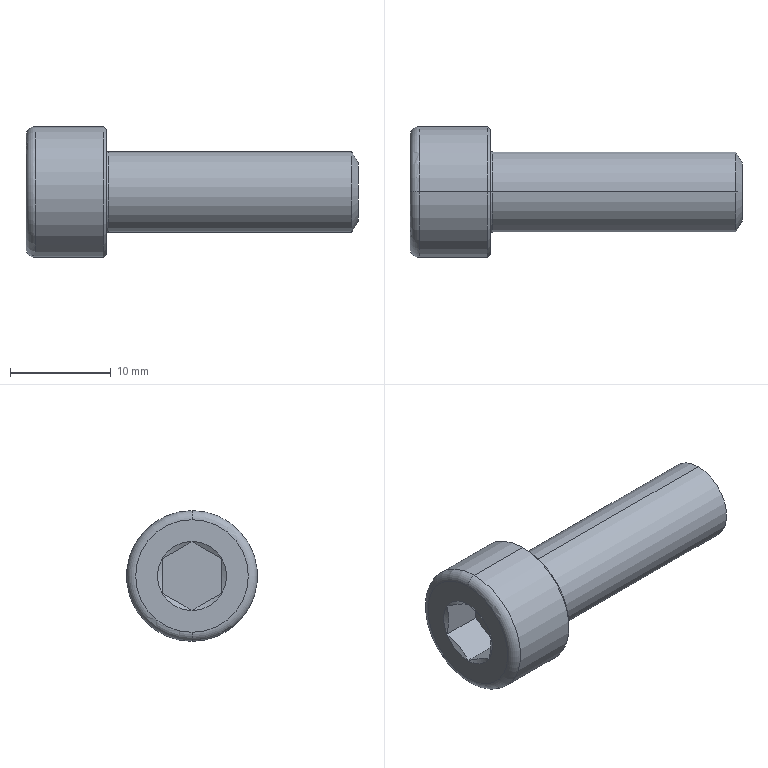Component | SolidWorks | M8_25_T70.1-1 | 1 solid | 28 faces | box 33 x 13 x 13 mm | volume 2179 mm3 | cone 10 | plane 10 | torus 4 | cylinder 4 | commonest cylinder face diameters 13 x2 8 x2 | material Plain Carbon Steel
STEP:
#1=COLOUR_RGB('',0.7922,0.8196,0.9333);
#2=FILL_AREA_STYLE_COLOUR('',#1);
#3=FILL_AREA_STYLE('',(#2));
#4=SURFACE_STYLE_FILL_AREA(#3);
#5=SURFACE_SIDE_STYLE('',(#4));
#6=SURFACE_STYLE_USAGE(.BOTH.,#5);
#7=PRESENTATION_STYLE_ASSIGNMENT((#6));
#8=CARTESIAN_POINT('',(-0.6339,1.67,1.426));
#9=VERTEX_POINT('',#8);
#10=CARTESIAN_POINT('',(-0.6339,1.67,1.914));
#11=VERTEX_POINT('',#10);
#12=CARTESIAN_POINT('',(-0.6339,1.67,1.67));
#13=DIRECTION('',(1.,0.,0.));
#14=DIRECTION('',(0.,0.,1.));
#15=AXIS2_PLACEMENT_3D('',#12,#13,#14);
#16=CIRCLE('',#15,0.2441);
#17=EDGE_CURVE('',#9,#11,#16,.T.);
#18=ORIENTED_EDGE('',*,*,#17,.F.);
#19=CARTESIAN_POINT('',(-0.6457,1.67,1.414));
#20=VERTEX_POINT('',#19);
#21=CARTESIAN_POINT('',(-0.6457,1.67,1.414));
#22=DIRECTION('',(-0.7071,0.,-0.7071));
#23=VECTOR('',#22,39.37);
#24=LINE('',#21,#23);
#25=EDGE_CURVE('',#9,#20,#24,.T.);
#26=ORIENTED_EDGE('',*,*,#25,.T.);
#27=CARTESIAN_POINT('',(-0.6457,1.67,1.926));
#28=VERTEX_POINT('',#27);
#29=CARTESIAN_POINT('',(-0.6457,1.67,1.67));
#30=DIRECTION('',(-1.,0.,0.));
#31=DIRECTION('',(0.,0.,1.));
#32=AXIS2_PLACEMENT_3D('',#29,#30,#31);
#33=CIRCLE('',#32,0.2559);
#34=EDGE_CURVE('',#28,#20,#33,.T.);
#35=ORIENTED_EDGE('',*,*,#34,.F.);
#36=CARTESIAN_POINT('',(-0.6457,1.67,1.926));
#37=DIRECTION('',(-0.7071,0.,0.7071));
#38=VECTOR('',#37,39.37);
#39=LINE('',#36,#38);
#40=EDGE_CURVE('',#11,#28,#39,.T.);
#41=ORIENTED_EDGE('',*,*,#40,.F.);
#42=EDGE_LOOP('',(#18,#26,#35,#41));
#43=FACE_OUTER_BOUND('',#42,.T.);
#44=CARTESIAN_POINT('',(-0.6457,1.67,1.67));
#45=DIRECTION('',(-1.,0.,0.));
#46=DIRECTION('',(0.,0.,1.));
#47=AXIS2_PLACEMENT_3D('',#44,#45,#46);
#48=CONICAL_SURFACE('',#47,0.2559,0.7854);
#49=ADVANCED_FACE('',(#43),#48,.T.);
#50=CARTESIAN_POINT('',(-0.9488,1.67,1.891));
#51=VERTEX_POINT('',#50);
#52=CARTESIAN_POINT('',(-0.9488,1.67,1.45));
#53=VERTEX_POINT('',#52);
#54=CARTESIAN_POINT('',(-0.9488,1.67,1.67));
#55=DIRECTION('',(-1.,0.,0.));
#56=DIRECTION('',(0.,0.,-1.));
#57=AXIS2_PLACEMENT_3D('',#54,#55,#56);
#58=CIRCLE('',#57,0.2205);
#59=EDGE_CURVE('',#51,#53,#58,.T.);
#60=ORIENTED_EDGE('',*,*,#59,.F.);
#61=CARTESIAN_POINT('',(-0.9134,1.67,1.926));
#62=VERTEX_POINT('',#61);
#63=CARTESIAN_POINT('',(-0.9134,1.67,1.891));
#64=DIRECTION('',(0.,1.,-0.));
#65=DIRECTION('',(0.,0.,1.));
#66=AXIS2_PLACEMENT_3D('',#63,#64,#65);
#67=CIRCLE('',#66,0.03543);
#68=EDGE_CURVE('',#51,#62,#67,.T.);
#69=ORIENTED_EDGE('',*,*,#68,.T.);
#70=CARTESIAN_POINT('',(-0.9134,1.67,1.414));
#71=VERTEX_POINT('',#70);
#72=CARTESIAN_POINT('',(-0.9134,1.67,1.67));
#73=DIRECTION('',(1.,0.,0.));
#74=DIRECTION('',(0.,0.,-1.));
#75=AXIS2_PLACEMENT_3D('',#72,#73,#74);
#76=CIRCLE('',#75,0.2559);
#77=EDGE_CURVE('',#71,#62,#76,.T.);
#78=ORIENTED_EDGE('',*,*,#77,.F.);
#79=CARTESIAN_POINT('',(-0.9134,1.67,1.45));
#80=DIRECTION('',(0.,-1.,0.));
#81=DIRECTION('',(0.,0.,-1.));
#82=AXIS2_PLACEMENT_3D('',#79,#80,#81);
#83=CIRCLE('',#82,0.03543);
#84=EDGE_CURVE('',#53,#71,#83,.T.);
#85=ORIENTED_EDGE('',*,*,#84,.F.);
#86=EDGE_LOOP('',(#60,#69,#78,#85));
#87=FACE_OUTER_BOUND('',#86,.T.);
#88=CARTESIAN_POINT('',(-0.9134,1.67,1.67));
#89=DIRECTION('',(1.,0.,0.));
#90=DIRECTION('',(0.,0.,-1.));
#91=AXIS2_PLACEMENT_3D('',#88,#89,#90);
#92=TOROIDAL_SURFACE('',#91,0.2205,0.03543);
#93=ADVANCED_FACE('',(#87),#92,.T.);
#94=CARTESIAN_POINT('',(0.3504,1.67,1.785));
#95=VERTEX_POINT('',#94);
#96=CARTESIAN_POINT('',(0.3504,1.67,1.555));
#97=VERTEX_POINT('',#96);
#98=CARTESIAN_POINT('',(0.3504,1.67,1.67));
#99=DIRECTION('',(-1.,0.,0.));
#100=DIRECTION('',(0.,0.,1.));
#101=AXIS2_PLACEMENT_3D('',#98,#99,#100);
#102=CIRCLE('',#101,0.1149);
#103=EDGE_CURVE('',#95,#97,#102,.T.);
#104=ORIENTED_EDGE('',*,*,#103,.T.);
#105=CARTESIAN_POINT('',(0.3258,1.67,1.513));
#106=VERTEX_POINT('',#105);
#107=CARTESIAN_POINT('',(0.3258,1.67,1.513));
#108=DIRECTION('',(-0.5,0.,-0.866));
#109=VECTOR('',#108,39.37);
#110=LINE('',#107,#109);
#111=EDGE_CURVE('',#97,#106,#110,.T.);
#112=ORIENTED_EDGE('',*,*,#111,.T.);
#113=CARTESIAN_POINT('',(0.3258,1.67,1.828));
#114=VERTEX_POINT('',#113);
#115=CARTESIAN_POINT('',(0.3258,1.67,1.67));
#116=DIRECTION('',(-1.,0.,0.));
#117=DIRECTION('',(0.,0.,1.));
#118=AXIS2_PLACEMENT_3D('',#115,#116,#117);
#119=CIRCLE('',#118,0.1575);
#120=EDGE_CURVE('',#114,#106,#119,.T.);
#121=ORIENTED_EDGE('',*,*,#120,.F.);
#122=CARTESIAN_POINT('',(0.3258,1.67,1.828));
#123=DIRECTION('',(-0.5,0.,0.866));
#124=VECTOR('',#123,39.37);
#125=LINE('',#122,#124);
#126=EDGE_CURVE('',#95,#114,#125,.T.);
#127=ORIENTED_EDGE('',*,*,#126,.F.);
#128=EDGE_LOOP('',(#104,#112,#121,#127));
#129=FACE_OUTER_BOUND('',#128,.T.);
#130=CARTESIAN_POINT('',(0.3258,1.67,1.67));
#131=DIRECTION('',(-1.,0.,0.));
#132=DIRECTION('',(0.,0.,1.));
#133=AXIS2_PLACEMENT_3D('',#130,#131,#132);
#134=CONICAL_SURFACE('',#133,0.1575,1.047);
#135=ADVANCED_FACE('',(#129),#134,.T.);
#136=CARTESIAN_POINT('',(-0.6339,1.67,1.505));
#137=VERTEX_POINT('',#136);
#138=CARTESIAN_POINT('',(-0.6339,1.67,1.836));
#139=VERTEX_POINT('',#138);
#140=CARTESIAN_POINT('',(-0.6339,1.67,1.67));
#141=DIRECTION('',(-1.,0.,0.));
#142=DIRECTION('',(0.,0.,1.));
#143=AXIS2_PLACEMENT_3D('',#140,#141,#142);
#144=CIRCLE('',#143,0.1654);
#145=EDGE_CURVE('',#137,#139,#144,.T.);
#146=ORIENTED_EDGE('',*,*,#145,.F.);
#147=CARTESIAN_POINT('',(-0.626,1.67,1.513));
#148=VERTEX_POINT('',#147);
#149=CARTESIAN_POINT('',(-0.626,1.67,1.505));
#150=DIRECTION('',(0.,1.,0.));
#151=DIRECTION('',(0.,0.,1.));
#152=AXIS2_PLACEMENT_3D('',#149,#150,#151);
#153=CIRCLE('',#152,0.007874);
#154=EDGE_CURVE('',#137,#148,#153,.T.);
#155=ORIENTED_EDGE('',*,*,#154,.T.);
#156=CARTESIAN_POINT('',(-0.626,1.67,1.828));
#157=VERTEX_POINT('',#156);
#158=CARTESIAN_POINT('',(-0.626,1.67,1.67));
#159=DIRECTION('',(-1.,0.,0.));
#160=DIRECTION('',(0.,0.,1.));
#161=AXIS2_PLACEMENT_3D('',#158,#159,#160);
#162=CIRCLE('',#161,0.1575);
#163=EDGE_CURVE('',#148,#157,#162,.T.);
#164=ORIENTED_EDGE('',*,*,#163,.T.);
#165=CARTESIAN_POINT('',(-0.626,1.67,1.836));
#166=DIRECTION('',(0.,-1.,0.));
#167=DIRECTION('',(0.,0.,-1.));
#168=AXIS2_PLACEMENT_3D('',#165,#166,#167);
#169=CIRCLE('',#168,0.007874);
#170=EDGE_CURVE('',#139,#157,#169,.T.);
#171=ORIENTED_EDGE('',*,*,#170,.F.);
#172=EDGE_LOOP('',(#146,#155,#164,#171));
#173=FACE_OUTER_BOUND('',#172,.T.);
#174=CARTESIAN_POINT('',(-0.626,1.67,1.67));
#175=DIRECTION('',(-1.,0.,0.));
#176=DIRECTION('',(0.,0.,1.));
#177=AXIS2_PLACEMENT_3D('',#174,#175,#176);
#178=TOROIDAL_SURFACE('',#177,0.1654,0.007874);
#179=ADVANCED_FACE('',(#173),#178,.F.);
#180=ORIENTED_EDGE('',*,*,#34,.T.);
#181=CARTESIAN_POINT('',(-0.9488,1.67,1.414));
#182=DIRECTION('',(-1.,0.,0.));
#183=VECTOR('',#182,39.37);
#184=LINE('',#181,#183);
#185=EDGE_CURVE('',#20,#71,#184,.T.);
#186=ORIENTED_EDGE('',*,*,#185,.T.);
#187=ORIENTED_EDGE('',*,*,#77,.T.);
#188=CARTESIAN_POINT('',(-0.9488,1.67,1.926));
#189=DIRECTION('',(-1.,0.,0.));
#190=VECTOR('',#189,39.37);
#191=LINE('',#188,#190);
#192=EDGE_CURVE('',#28,#62,#191,.T.);
#193=ORIENTED_EDGE('',*,*,#192,.F.);
#194=EDGE_LOOP('',(#180,#186,#187,#193));
#195=FACE_OUTER_BOUND('',#194,.T.);
#196=CARTESIAN_POINT('',(-0.9488,1.67,1.67));
#197=DIRECTION('',(-1.,0.,0.));
#198=DIRECTION('',(0.,0.,1.));
#199=AXIS2_PLACEMENT_3D('',#196,#197,#198);
#200=CYLINDRICAL_SURFACE('',#199,0.2559);
#201=ADVANCED_FACE('',(#195),#200,.T.);
#202=ORIENTED_EDGE('',*,*,#120,.T.);
#203=CARTESIAN_POINT('',(-0.9488,1.67,1.513));
#204=DIRECTION('',(-1.,0.,0.));
#205=VECTOR('',#204,39.37);
#206=LINE('',#203,#205);
#207=EDGE_CURVE('',#106,#148,#206,.T.);
#208=ORIENTED_EDGE('',*,*,#207,.T.);
#209=CARTESIAN_POINT('',(-0.626,1.67,1.67));
#210=DIRECTION('',(-1.,0.,0.));
#211=DIRECTION('',(0.,0.,1.));
#212=AXIS2_PLACEMENT_3D('',#209,#210,#211);
#213=CIRCLE('',#212,0.1575);
#214=EDGE_CURVE('',#157,#148,#213,.T.);
#215=ORIENTED_EDGE('',*,*,#214,.F.);
#216=CARTESIAN_POINT('',(-0.9488,1.67,1.828));
#217=DIRECTION('',(-1.,0.,0.));
#218=VECTOR('',#217,39.37);
#219=LINE('',#216,#218);
#220=EDGE_CURVE('',#114,#157,#219,.T.);
#221=ORIENTED_EDGE('',*,*,#220,.F.);
#222=EDGE_LOOP('',(#202,#208,#215,#221));
#223=FACE_OUTER_BOUND('',#222,.T.);
#224=CARTESIAN_POINT('',(-0.9488,1.67,1.67));
#225=DIRECTION('',(-1.,0.,0.));
#226=DIRECTION('',(0.,0.,1.));
#227=AXIS2_PLACEMENT_3D('',#224,#225,#226);
#228=CYLINDRICAL_SURFACE('',#227,0.1575);
#229=ADVANCED_FACE('',(#223),#228,.T.);
#230=ORIENTED_EDGE('',*,*,#207,.F.);
#231=CARTESIAN_POINT('',(0.3258,1.67,1.67));
#232=DIRECTION('',(-1.,0.,0.));
#233=DIRECTION('',(0.,0.,1.));
#234=AXIS2_PLACEMENT_3D('',#231,#232,#233);
#235=CIRCLE('',#234,0.1575);
#236=EDGE_CURVE('',#106,#114,#235,.T.);
#237=ORIENTED_EDGE('',*,*,#236,.T.);
#238=ORIENTED_EDGE('',*,*,#220,.T.);
#239=ORIENTED_EDGE('',*,*,#163,.F.);
#240=EDGE_LOOP('',(#230,#237,#238,#239));
#241=FACE_OUTER_BOUND('',#240,.T.);
#242=CARTESIAN_POINT('',(-0.9488,1.67,1.67));
#243=DIRECTION('',(-1.,0.,0.));
#244=DIRECTION('',(0.,0.,1.));
#245=AXIS2_PLACEMENT_3D('',#242,#243,#244);
#246=CYLINDRICAL_SURFACE('',#245,0.1575);
#247=ADVANCED_FACE('',(#241),#246,.T.);
#248=CARTESIAN_POINT('',(-0.9488,1.67,1.67));
#249=DIRECTION('',(-1.,0.,0.));
#250=DIRECTION('',(0.,0.,-1.));
#251=AXIS2_PLACEMENT_3D('',#248,#249,#250);
#252=CIRCLE('',#251,0.2205);
#253=EDGE_CURVE('',#53,#51,#252,.T.);
#254=ORIENTED_EDGE('',*,*,#253,.T.);
#255=ORIENTED_EDGE('',*,*,#59,.T.);
#256=EDGE_LOOP('',(#254,#255));
#257=FACE_OUTER_BOUND('',#256,.T.);
#258=CARTESIAN_POINT('',(-0.9488,1.67,1.535));
#259=VERTEX_POINT('',#258);
#260=CARTESIAN_POINT('',(-0.9488,1.553,1.603));
#261=VERTEX_POINT('',#260);
#262=CARTESIAN_POINT('',(-0.9488,1.67,1.67));
#263=DIRECTION('',(-1.,0.,0.));
#264=DIRECTION('',(0.,0.,1.));
#265=AXIS2_PLACEMENT_3D('',#262,#263,#264);
#266=CIRCLE('',#265,0.135);
#267=EDGE_CURVE('',#259,#261,#266,.T.);
#268=ORIENTED_EDGE('',*,*,#267,.F.);
#269=CARTESIAN_POINT('',(-0.9488,1.787,1.603));
#270=VERTEX_POINT('',#269);
#271=CARTESIAN_POINT('',(-0.9488,1.67,1.67));
#272=DIRECTION('',(-1.,0.,0.));
#273=DIRECTION('',(0.,0.,1.));
#274=AXIS2_PLACEMENT_3D('',#271,#272,#273);
#275=CIRCLE('',#274,0.135);
#276=EDGE_CURVE('',#270,#259,#275,.T.);
#277=ORIENTED_EDGE('',*,*,#276,.F.);
#278=CARTESIAN_POINT('',(-0.9488,1.787,1.738));
#279=VERTEX_POINT('',#278);
#280=CARTESIAN_POINT('',(-0.9488,1.67,1.67));
#281=DIRECTION('',(-1.,0.,0.));
#282=DIRECTION('',(0.,0.,1.));
#283=AXIS2_PLACEMENT_3D('',#280,#281,#282);
#284=CIRCLE('',#283,0.135);
#285=EDGE_CURVE('',#279,#270,#284,.T.);
#286=ORIENTED_EDGE('',*,*,#285,.F.);
#287=CARTESIAN_POINT('',(-0.9488,1.67,1.805));
#288=VERTEX_POINT('',#287);
#289=CARTESIAN_POINT('',(-0.9488,1.67,1.67));
#290=DIRECTION('',(-1.,0.,0.));
#291=DIRECTION('',(0.,0.,1.));
#292=AXIS2_PLACEMENT_3D('',#289,#290,#291);
#293=CIRCLE('',#292,0.135);
#294=EDGE_CURVE('',#288,#279,#293,.T.);
#295=ORIENTED_EDGE('',*,*,#294,.F.);
#296=CARTESIAN_POINT('',(-0.9488,1.553,1.738));
#297=VERTEX_POINT('',#296);
#298=CARTESIAN_POINT('',(-0.9488,1.67,1.67));
#299=DIRECTION('',(-1.,0.,0.));
#300=DIRECTION('',(0.,0.,1.));
#301=AXIS2_PLACEMENT_3D('',#298,#299,#300);
#302=CIRCLE('',#301,0.135);
#303=EDGE_CURVE('',#297,#288,#302,.T.);
#304=ORIENTED_EDGE('',*,*,#303,.F.);
#305=CARTESIAN_POINT('',(-0.9488,1.67,1.67));
#306=DIRECTION('',(-1.,0.,0.));
#307=DIRECTION('',(0.,0.,1.));
#308=AXIS2_PLACEMENT_3D('',#305,#306,#307);
#309=CIRCLE('',#308,0.135);
#310=EDGE_CURVE('',#261,#297,#309,.T.);
#311=ORIENTED_EDGE('',*,*,#310,.F.);
#312=EDGE_LOOP('',(#268,#277,#286,#295,#304,#311));
#313=FACE_BOUND('',#312,.T.);
#314=CARTESIAN_POINT('',(-0.9488,1.67,1.67));
#315=DIRECTION('',(1.,0.,0.));
#316=DIRECTION('',(0.,0.,-1.));
#317=AXIS2_PLACEMENT_3D('',#314,#315,#316);
#318=PLANE('',#317);
#319=ADVANCED_FACE('',(#257,#313),#318,.F.);
#320=ORIENTED_EDGE('',*,*,#185,.F.);
#321=CARTESIAN_POINT('',(-0.6457,1.67,1.67));
#322=DIRECTION('',(-1.,0.,0.));
#323=DIRECTION('',(0.,0.,1.));
#324=AXIS2_PLACEMENT_3D('',#321,#322,#323);
#325=CIRCLE('',#324,0.2559);
#326=EDGE_CURVE('',#20,#28,#325,.T.);
#327=ORIENTED_EDGE('',*,*,#326,.T.);
#328=ORIENTED_EDGE('',*,*,#192,.T.);
#329=CARTESIAN_POINT('',(-0.9134,1.67,1.67));
#330=DIRECTION('',(1.,0.,0.));
#331=DIRECTION('',(0.,0.,-1.));
#332=AXIS2_PLACEMENT_3D('',#329,#330,#331);
#333=CIRCLE('',#332,0.2559);
#334=EDGE_CURVE('',#62,#71,#333,.T.);
#335=ORIENTED_EDGE('',*,*,#334,.T.);
#336=EDGE_LOOP('',(#320,#327,#328,#335));
#337=FACE_OUTER_BOUND('',#336,.T.);
#338=CARTESIAN_POINT('',(-0.9488,1.67,1.67));
#339=DIRECTION('',(-1.,0.,0.));
#340=DIRECTION('',(0.,0.,1.));
#341=AXIS2_PLACEMENT_3D('',#338,#339,#340);
#342=CYLINDRICAL_SURFACE('',#341,0.2559);
#343=ADVANCED_FACE('',(#337),#342,.T.);
#344=CARTESIAN_POINT('',(-0.6339,1.67,1.67));
#345=DIRECTION('',(1.,0.,0.));
#346=DIRECTION('',(0.,0.,1.));
#347=AXIS2_PLACEMENT_3D('',#344,#345,#346);
#348=CIRCLE('',#347,0.2441);
#349=EDGE_CURVE('',#11,#9,#348,.T.);
#350=ORIENTED_EDGE('',*,*,#349,.T.);
#351=ORIENTED_EDGE('',*,*,#17,.T.);
#352=EDGE_LOOP('',(#350,#351));
#353=FACE_OUTER_BOUND('',#352,.T.);
#354=CARTESIAN_POINT('',(-0.6339,1.67,1.67));
#355=DIRECTION('',(-1.,0.,0.));
#356=DIRECTION('',(0.,0.,1.));
#357=AXIS2_PLACEMENT_3D('',#354,#355,#356);
#358=CIRCLE('',#357,0.1654);
#359=EDGE_CURVE('',#139,#137,#358,.T.);
#360=ORIENTED_EDGE('',*,*,#359,.T.);
#361=ORIENTED_EDGE('',*,*,#145,.T.);
#362=EDGE_LOOP('',(#360,#361));
#363=FACE_BOUND('',#362,.T.);
#364=CARTESIAN_POINT('',(-0.6339,1.926,1.67));
#365=DIRECTION('',(-1.,0.,0.));
#366=DIRECTION('',(0.,0.,1.));
#367=AXIS2_PLACEMENT_3D('',#364,#365,#366);
#368=PLANE('',#367);
#369=ADVANCED_FACE('',(#353,#363),#368,.F.);
#370=ORIENTED_EDGE('',*,*,#154,.F.);
#371=ORIENTED_EDGE('',*,*,#359,.F.);
#372=ORIENTED_EDGE('',*,*,#170,.T.);
#373=ORIENTED_EDGE('',*,*,#214,.T.);
#374=EDGE_LOOP('',(#370,#371,#372,#373));
#375=FACE_OUTER_BOUND('',#374,.T.);
#376=CARTESIAN_POINT('',(-0.626,1.67,1.67));
#377=DIRECTION('',(-1.,0.,0.));
#378=DIRECTION('',(0.,0.,1.));
#379=AXIS2_PLACEMENT_3D('',#376,#377,#378);
#380=TOROIDAL_SURFACE('',#379,0.1654,0.007874);
#381=ADVANCED_FACE('',(#375),#380,.F.);
#382=ORIENTED_EDGE('',*,*,#111,.F.);
#383=CARTESIAN_POINT('',(0.3504,1.67,1.67));
#384=DIRECTION('',(-1.,0.,0.));
#385=DIRECTION('',(0.,0.,1.));
#386=AXIS2_PLACEMENT_3D('',#383,#384,#385);
#387=CIRCLE('',#386,0.1149);
#388=EDGE_CURVE('',#97,#95,#387,.T.);
#389=ORIENTED_EDGE('',*,*,#388,.T.);
#390=ORIENTED_EDGE('',*,*,#126,.T.);
#391=ORIENTED_EDGE('',*,*,#236,.F.);
#392=EDGE_LOOP('',(#382,#389,#390,#391));
#393=FACE_OUTER_BOUND('',#392,.T.);
#394=CARTESIAN_POINT('',(0.3258,1.67,1.67));
#395=DIRECTION('',(-1.,0.,0.));
#396=DIRECTION('',(0.,0.,1.));
#397=AXIS2_PLACEMENT_3D('',#394,#395,#396);
#398=CONICAL_SURFACE('',#397,0.1575,1.047);
#399=ADVANCED_FACE('',(#393),#398,.T.);
#400=ORIENTED_EDGE('',*,*,#103,.F.);
#401=ORIENTED_EDGE('',*,*,#388,.F.);
#402=EDGE_LOOP('',(#400,#401));
#403=FACE_OUTER_BOUND('',#402,.T.);
#404=CARTESIAN_POINT('',(0.3504,1.828,1.67));
#405=DIRECTION('',(-1.,0.,0.));
#406=DIRECTION('',(0.,0.,1.));
#407=AXIS2_PLACEMENT_3D('',#404,#405,#406);
#408=PLANE('',#407);
#409=ADVANCED_FACE('',(#403),#408,.F.);
#410=ORIENTED_EDGE('',*,*,#68,.F.);
#411=ORIENTED_EDGE('',*,*,#253,.F.);
#412=ORIENTED_EDGE('',*,*,#84,.T.);
#413=ORIENTED_EDGE('',*,*,#334,.F.);
#414=EDGE_LOOP('',(#410,#411,#412,#413));
#415=FACE_OUTER_BOUND('',#414,.T.);
#416=CARTESIAN_POINT('',(-0.9134,1.67,1.67));
#417=DIRECTION('',(1.,0.,0.));
#418=DIRECTION('',(0.,0.,-1.));
#419=AXIS2_PLACEMENT_3D('',#416,#417,#418);
#420=TOROIDAL_SURFACE('',#419,0.2205,0.03543);
#421=ADVANCED_FACE('',(#415),#420,.T.);
#422=ORIENTED_EDGE('',*,*,#25,.F.);
#423=ORIENTED_EDGE('',*,*,#349,.F.);
#424=ORIENTED_EDGE('',*,*,#40,.T.);
#425=ORIENTED_EDGE('',*,*,#326,.F.);
#426=EDGE_LOOP('',(#422,#423,#424,#425));
#427=FACE_OUTER_BOUND('',#426,.T.);
#428=CARTESIAN_POINT('',(-0.6457,1.67,1.67));
#429=DIRECTION('',(-1.,0.,0.));
#430=DIRECTION('',(0.,0.,1.));
#431=AXIS2_PLACEMENT_3D('',#428,#429,#430);
#432=CONICAL_SURFACE('',#431,0.2559,0.7854);
#433=ADVANCED_FACE('',(#427),#432,.T.);
#434=ORIENTED_EDGE('',*,*,#294,.T.);
#435=CARTESIAN_POINT('',(-0.9488,1.67,1.805));
#436=CARTESIAN_POINT('',(-0.9425,1.689,1.794));
#437=CARTESIAN_POINT('',(-0.9384,1.709,1.783));
#438=CARTESIAN_POINT('',(-0.9384,1.739,1.766));
#439=CARTESIAN_POINT('',(-0.9394,1.749,1.76));
#440=CARTESIAN_POINT('',(-0.943,1.768,1.749));
#441=CARTESIAN_POINT('',(-0.9456,1.778,1.743));
#442=CARTESIAN_POINT('',(-0.9488,1.787,1.738));
#443=B_SPLINE_CURVE_WITH_KNOTS('',3,(#435,#436,#437,#438,#439,#440,#441,#442),.UNSPECIFIED.,.F.,.F.,(4,2,2,4),(0.00000024,0.001732,0.002598,0.003464),.UNSPECIFIED.);
#444=EDGE_CURVE('',#288,#279,#443,.T.);
#445=ORIENTED_EDGE('',*,*,#444,.F.);
#446=EDGE_LOOP('',(#434,#445));
#447=FACE_OUTER_BOUND('',#446,.T.);
#448=CARTESIAN_POINT('',(-0.9488,1.67,1.67));
#449=DIRECTION('',(-1.,0.,0.));
#450=DIRECTION('',(0.,0.,1.));
#451=AXIS2_PLACEMENT_3D('',#448,#449,#450);
#452=CONICAL_SURFACE('',#451,0.135,1.047);
#453=ADVANCED_FACE('',(#447),#452,.F.);
#454=ORIENTED_EDGE('',*,*,#285,.T.);
#455=CARTESIAN_POINT('',(-0.9488,1.787,1.738));
#456=CARTESIAN_POINT('',(-0.9457,1.787,1.727));
#457=CARTESIAN_POINT('',(-0.943,1.787,1.716));
#458=CARTESIAN_POINT('',(-0.9394,1.787,1.693));
#459=CARTESIAN_POINT('',(-0.9384,1.787,1.682));
#460=CARTESIAN_POINT('',(-0.9384,1.787,1.659));
#461=CARTESIAN_POINT('',(-0.9394,1.787,1.648));
#462=CARTESIAN_POINT('',(-0.943,1.787,1.625));
#463=CARTESIAN_POINT('',(-0.9457,1.787,1.614));
#464=CARTESIAN_POINT('',(-0.9488,1.787,1.603));
#465=B_SPLINE_CURVE_WITH_KNOTS('',3,(#455,#456,#457,#458,#459,#460,#461,#462,#463,#464),.UNSPECIFIED.,.F.,.F.,(4,2,2,2,4),(0.009185,0.01005,0.01092,0.01179,0.01266),.UNSPECIFIED.);
#466=EDGE_CURVE('',#279,#270,#465,.T.);
#467=ORIENTED_EDGE('',*,*,#466,.F.);
#468=EDGE_LOOP('',(#454,#467));
#469=FACE_OUTER_BOUND('',#468,.T.);
#470=CARTESIAN_POINT('',(-0.9488,1.67,1.67));
#471=DIRECTION('',(-1.,0.,0.));
#472=DIRECTION('',(0.,0.,1.));
#473=AXIS2_PLACEMENT_3D('',#470,#471,#472);
#474=CONICAL_SURFACE('',#473,0.135,1.047);
#475=ADVANCED_FACE('',(#469),#474,.F.);
#476=ORIENTED_EDGE('',*,*,#276,.T.);
#477=CARTESIAN_POINT('',(-0.9488,1.787,1.603));
#478=CARTESIAN_POINT('',(-0.9425,1.768,1.592));
#479=CARTESIAN_POINT('',(-0.9384,1.749,1.581));
#480=CARTESIAN_POINT('',(-0.9384,1.719,1.563));
#481=CARTESIAN_POINT('',(-0.9394,1.709,1.558));
#482=CARTESIAN_POINT('',(-0.943,1.69,1.546));
#483=CARTESIAN_POINT('',(-0.9456,1.68,1.541));
#484=CARTESIAN_POINT('',(-0.9488,1.67,1.535));
#485=B_SPLINE_CURVE_WITH_KNOTS('',3,(#477,#478,#479,#480,#481,#482,#483,#484),.UNSPECIFIED.,.F.,.F.,(4,2,2,4),(0.00000024,0.001732,0.002598,0.003464),.UNSPECIFIED.);
#486=EDGE_CURVE('',#270,#259,#485,.T.);
#487=ORIENTED_EDGE('',*,*,#486,.F.);
#488=EDGE_LOOP('',(#476,#487));
#489=FACE_OUTER_BOUND('',#488,.T.);
#490=CARTESIAN_POINT('',(-0.9488,1.67,1.67));
#491=DIRECTION('',(-1.,0.,0.));
#492=DIRECTION('',(0.,0.,1.));
#493=AXIS2_PLACEMENT_3D('',#490,#491,#492);
#494=CONICAL_SURFACE('',#493,0.135,1.047);
#495=ADVANCED_FACE('',(#489),#494,.F.);
#496=ORIENTED_EDGE('',*,*,#267,.T.);
#497=CARTESIAN_POINT('',(-0.9488,1.67,1.535));
#498=CARTESIAN_POINT('',(-0.9425,1.651,1.546));
#499=CARTESIAN_POINT('',(-0.9384,1.632,1.558));
#500=CARTESIAN_POINT('',(-0.9384,1.602,1.575));
#501=CARTESIAN_POINT('',(-0.9394,1.592,1.58));
#502=CARTESIAN_POINT('',(-0.943,1.573,1.592));
#503=CARTESIAN_POINT('',(-0.9456,1.563,1.597));
#504=CARTESIAN_POINT('',(-0.9488,1.553,1.603));
#505=B_SPLINE_CURVE_WITH_KNOTS('',3,(#497,#498,#499,#500,#501,#502,#503,#504),.UNSPECIFIED.,.F.,.F.,(4,2,2,4),(0.00000024,0.001732,0.002598,0.003464),.UNSPECIFIED.);
#506=EDGE_CURVE('',#259,#261,#505,.T.);
#507=ORIENTED_EDGE('',*,*,#506,.F.);
#508=EDGE_LOOP('',(#496,#507));
#509=FACE_OUTER_BOUND('',#508,.T.);
#510=CARTESIAN_POINT('',(-0.9488,1.67,1.67));
#511=DIRECTION('',(-1.,0.,0.));
#512=DIRECTION('',(0.,0.,1.));
#513=AXIS2_PLACEMENT_3D('',#510,#511,#512);
#514=CONICAL_SURFACE('',#513,0.135,1.047);
#515=ADVANCED_FACE('',(#509),#514,.F.);
#516=ORIENTED_EDGE('',*,*,#310,.T.);
#517=CARTESIAN_POINT('',(-0.9488,1.553,1.603));
#518=CARTESIAN_POINT('',(-0.9457,1.553,1.614));
#519=CARTESIAN_POINT('',(-0.943,1.553,1.625));
#520=CARTESIAN_POINT('',(-0.9394,1.553,1.648));
#521=CARTESIAN_POINT('',(-0.9384,1.553,1.659));
#522=CARTESIAN_POINT('',(-0.9384,1.553,1.682));
#523=CARTESIAN_POINT('',(-0.9394,1.553,1.693));
#524=CARTESIAN_POINT('',(-0.943,1.553,1.716));
#525=CARTESIAN_POINT('',(-0.9457,1.553,1.727));
#526=CARTESIAN_POINT('',(-0.9488,1.553,1.738));
#527=B_SPLINE_CURVE_WITH_KNOTS('',3,(#517,#518,#519,#520,#521,#522,#523,#524,#525,#526),.UNSPECIFIED.,.F.,.F.,(4,2,2,2,4),(0.002941,0.003808,0.004675,0.005542,0.006409),.UNSPECIFIED.);
#528=EDGE_CURVE('',#261,#297,#527,.T.);
#529=ORIENTED_EDGE('',*,*,#528,.F.);
#530=EDGE_LOOP('',(#516,#529));
#531=FACE_OUTER_BOUND('',#530,.T.);
#532=CARTESIAN_POINT('',(-0.9488,1.67,1.67));
#533=DIRECTION('',(-1.,0.,0.));
#534=DIRECTION('',(0.,0.,1.));
#535=AXIS2_PLACEMENT_3D('',#532,#533,#534);
#536=CONICAL_SURFACE('',#535,0.135,1.047);
#537=ADVANCED_FACE('',(#531),#536,.F.);
#538=ORIENTED_EDGE('',*,*,#303,.T.);
#539=CARTESIAN_POINT('',(-0.9488,1.553,1.738));
#540=CARTESIAN_POINT('',(-0.9425,1.572,1.749));
#541=CARTESIAN_POINT('',(-0.9384,1.592,1.76));
#542=CARTESIAN_POINT('',(-0.9384,1.622,1.777));
#543=CARTESIAN_POINT('',(-0.9394,1.632,1.783));
#544=CARTESIAN_POINT('',(-0.943,1.651,1.794));
#545=CARTESIAN_POINT('',(-0.9456,1.661,1.8));
#546=CARTESIAN_POINT('',(-0.9488,1.67,1.805));
#547=B_SPLINE_CURVE_WITH_KNOTS('',3,(#539,#540,#541,#542,#543,#544,#545,#546),.UNSPECIFIED.,.F.,.F.,(4,2,2,4),(0.00000024,0.001732,0.002598,0.003464),.UNSPECIFIED.);
#548=EDGE_CURVE('',#297,#288,#547,.T.);
#549=ORIENTED_EDGE('',*,*,#548,.F.);
#550=EDGE_LOOP('',(#538,#549));
#551=FACE_OUTER_BOUND('',#550,.T.);
#552=CARTESIAN_POINT('',(-0.9488,1.67,1.67));
#553=DIRECTION('',(-1.,0.,0.));
#554=DIRECTION('',(0.,0.,1.));
#555=AXIS2_PLACEMENT_3D('',#552,#553,#554);
#556=CONICAL_SURFACE('',#555,0.135,1.047);
#557=ADVANCED_FACE('',(#551),#556,.F.);
#558=CARTESIAN_POINT('',(-0.7913,1.553,1.738));
#559=VERTEX_POINT('',#558);
#560=CARTESIAN_POINT('',(-0.7913,1.67,1.805));
#561=VERTEX_POINT('',#560);
#562=CARTESIAN_POINT('',(-0.7913,1.553,1.738));
#563=DIRECTION('',(0.,0.866,0.5));
#564=VECTOR('',#563,39.37);
#565=LINE('',#562,#564);
#566=EDGE_CURVE('',#559,#561,#565,.T.);
#567=ORIENTED_EDGE('',*,*,#566,.T.);
#568=CARTESIAN_POINT('',(-0.7913,1.787,1.738));
#569=VERTEX_POINT('',#568);
#570=CARTESIAN_POINT('',(-0.7913,1.67,1.805));
#571=DIRECTION('',(0.,0.866,-0.5));
#572=VECTOR('',#571,39.37);
#573=LINE('',#570,#572);
#574=EDGE_CURVE('',#561,#569,#573,.T.);
#575=ORIENTED_EDGE('',*,*,#574,.T.);
#576=CARTESIAN_POINT('',(-0.7913,1.787,1.603));
#577=VERTEX_POINT('',#576);
#578=CARTESIAN_POINT('',(-0.7913,1.787,1.738));
#579=DIRECTION('',(0.,0.,-1.));
#580=VECTOR('',#579,39.37);
#581=LINE('',#578,#580);
#582=EDGE_CURVE('',#569,#577,#581,.T.);
#583=ORIENTED_EDGE('',*,*,#582,.T.);
#584=CARTESIAN_POINT('',(-0.7913,1.67,1.535));
#585=VERTEX_POINT('',#584);
#586=CARTESIAN_POINT('',(-0.7913,1.787,1.603));
#587=DIRECTION('',(0.,-0.866,-0.5));
#588=VECTOR('',#587,39.37);
#589=LINE('',#586,#588);
#590=EDGE_CURVE('',#577,#585,#589,.T.);
#591=ORIENTED_EDGE('',*,*,#590,.T.);
#592=CARTESIAN_POINT('',(-0.7913,1.553,1.603));
#593=VERTEX_POINT('',#592);
#594=CARTESIAN_POINT('',(-0.7913,1.67,1.535));
#595=DIRECTION('',(0.,-0.866,0.5));
#596=VECTOR('',#595,39.37);
#597=LINE('',#594,#596);
#598=EDGE_CURVE('',#585,#593,#597,.T.);
#599=ORIENTED_EDGE('',*,*,#598,.T.);
#600=CARTESIAN_POINT('',(-0.7913,1.553,1.603));
#601=DIRECTION('',(0.,-0.,1.));
#602=VECTOR('',#601,39.37);
#603=LINE('',#600,#602);
#604=EDGE_CURVE('',#593,#559,#603,.T.);
#605=ORIENTED_EDGE('',*,*,#604,.T.);
#606=EDGE_LOOP('',(#567,#575,#583,#591,#599,#605));
#607=FACE_OUTER_BOUND('',#606,.T.);
#608=CARTESIAN_POINT('',(-0.7913,1.553,1.738));
#609=DIRECTION('',(1.,0.,0.));
#610=DIRECTION('',(0.,0.,-1.));
#611=AXIS2_PLACEMENT_3D('',#608,#609,#610);
#612=PLANE('',#611);
#613=ADVANCED_FACE('',(#607),#612,.F.);
#614=CARTESIAN_POINT('',(-0.7913,1.67,1.805));
#615=DIRECTION('',(-1.,0.,0.));
#616=VECTOR('',#615,39.37);
#617=LINE('',#614,#616);
#618=EDGE_CURVE('',#561,#288,#617,.T.);
#619=ORIENTED_EDGE('',*,*,#618,.T.);
#620=ORIENTED_EDGE('',*,*,#444,.T.);
#621=CARTESIAN_POINT('',(-0.7913,1.787,1.738));
#622=DIRECTION('',(-1.,0.,0.));
#623=VECTOR('',#622,39.37);
#624=LINE('',#621,#623);
#625=EDGE_CURVE('',#569,#279,#624,.T.);
#626=ORIENTED_EDGE('',*,*,#625,.F.);
#627=ORIENTED_EDGE('',*,*,#574,.F.);
#628=EDGE_LOOP('',(#619,#620,#626,#627));
#629=FACE_OUTER_BOUND('',#628,.T.);
#630=CARTESIAN_POINT('',(-0.7913,1.67,1.805));
#631=DIRECTION('',(0.,0.5,0.866));
#632=DIRECTION('',(0.,-0.866,0.5));
#633=AXIS2_PLACEMENT_3D('',#630,#631,#632);
#634=PLANE('',#633);
#635=ADVANCED_FACE('',(#629),#634,.F.);
#636=ORIENTED_EDGE('',*,*,#625,.T.);
#637=ORIENTED_EDGE('',*,*,#466,.T.);
#638=CARTESIAN_POINT('',(-0.7913,1.787,1.603));
#639=DIRECTION('',(-1.,0.,0.));
#640=VECTOR('',#639,39.37);
#641=LINE('',#638,#640);
#642=EDGE_CURVE('',#577,#270,#641,.T.);
#643=ORIENTED_EDGE('',*,*,#642,.F.);
#644=ORIENTED_EDGE('',*,*,#582,.F.);
#645=EDGE_LOOP('',(#636,#637,#643,#644));
#646=FACE_OUTER_BOUND('',#645,.T.);
#647=CARTESIAN_POINT('',(-0.7913,1.787,1.738));
#648=DIRECTION('',(0.,1.,0.));
#649=DIRECTION('',(0.,0.,1.));
#650=AXIS2_PLACEMENT_3D('',#647,#648,#649);
#651=PLANE('',#650);
#652=ADVANCED_FACE('',(#646),#651,.F.);
#653=ORIENTED_EDGE('',*,*,#642,.T.);
#654=ORIENTED_EDGE('',*,*,#486,.T.);
#655=CARTESIAN_POINT('',(-0.7913,1.67,1.535));
#656=DIRECTION('',(-1.,0.,0.));
#657=VECTOR('',#656,39.37);
#658=LINE('',#655,#657);
#659=EDGE_CURVE('',#585,#259,#658,.T.);
#660=ORIENTED_EDGE('',*,*,#659,.F.);
#661=ORIENTED_EDGE('',*,*,#590,.F.);
#662=EDGE_LOOP('',(#653,#654,#660,#661));
#663=FACE_OUTER_BOUND('',#662,.T.);
#664=CARTESIAN_POINT('',(-0.7913,1.787,1.603));
#665=DIRECTION('',(0.,0.5,-0.866));
#666=DIRECTION('',(0.,0.866,0.5));
#667=AXIS2_PLACEMENT_3D('',#664,#665,#666);
#668=PLANE('',#667);
#669=ADVANCED_FACE('',(#663),#668,.F.);
#670=ORIENTED_EDGE('',*,*,#659,.T.);
#671=ORIENTED_EDGE('',*,*,#506,.T.);
#672=CARTESIAN_POINT('',(-0.7913,1.553,1.603));
#673=DIRECTION('',(-1.,0.,0.));
#674=VECTOR('',#673,39.37);
#675=LINE('',#672,#674);
#676=EDGE_CURVE('',#593,#261,#675,.T.);
#677=ORIENTED_EDGE('',*,*,#676,.F.);
#678=ORIENTED_EDGE('',*,*,#598,.F.);
#679=EDGE_LOOP('',(#670,#671,#677,#678));
#680=FACE_OUTER_BOUND('',#679,.T.);
#681=CARTESIAN_POINT('',(-0.7913,1.67,1.535));
#682=DIRECTION('',(0.,-0.5,-0.866));
#683=DIRECTION('',(0.,0.866,-0.5));
#684=AXIS2_PLACEMENT_3D('',#681,#682,#683);
#685=PLANE('',#684);
#686=ADVANCED_FACE('',(#680),#685,.F.);
#687=ORIENTED_EDGE('',*,*,#676,.T.);
#688=ORIENTED_EDGE('',*,*,#528,.T.);
#689=CARTESIAN_POINT('',(-0.7913,1.553,1.738));
#690=DIRECTION('',(-1.,0.,0.));
#691=VECTOR('',#690,39.37);
#692=LINE('',#689,#691);
#693=EDGE_CURVE('',#559,#297,#692,.T.);
#694=ORIENTED_EDGE('',*,*,#693,.F.);
#695=ORIENTED_EDGE('',*,*,#604,.F.);
#696=EDGE_LOOP('',(#687,#688,#694,#695));
#697=FACE_OUTER_BOUND('',#696,.T.);
#698=CARTESIAN_POINT('',(-0.7913,1.553,1.603));
#699=DIRECTION('',(0.,-1.,-0.));
#700=DIRECTION('',(0.,0.,-1.));
#701=AXIS2_PLACEMENT_3D('',#698,#699,#700);
#702=PLANE('',#701);
#703=ADVANCED_FACE('',(#697),#702,.F.);
#704=ORIENTED_EDGE('',*,*,#693,.T.);
#705=ORIENTED_EDGE('',*,*,#548,.T.);
#706=ORIENTED_EDGE('',*,*,#618,.F.);
#707=ORIENTED_EDGE('',*,*,#566,.F.);
#708=EDGE_LOOP('',(#704,#705,#706,#707));
#709=FACE_OUTER_BOUND('',#708,.T.);
#710=CARTESIAN_POINT('',(-0.7913,1.553,1.738));
#711=DIRECTION('',(0.,-0.5,0.866));
#712=DIRECTION('',(0.,-0.866,-0.5));
#713=AXIS2_PLACEMENT_3D('',#710,#711,#712);
#714=PLANE('',#713);
#715=ADVANCED_FACE('',(#709),#714,.F.);
#716=CLOSED_SHELL('',(#49,#93,#135,#179,#201,#229,#247,#319,#343,#369,#381,#399,#409,#421,#433,#453,#475,#495,#515,#537,#557,#613,#635,#652,#669,#686,#703,#715));
#717=MANIFOLD_SOLID_BREP('',#716);
#718=STYLED_ITEM('',(#7),#717);
#719=PRESENTATION_LAYER_ASSIGNMENT('','',(#718));
#720=(LENGTH_UNIT()NAMED_UNIT(*)SI_UNIT($,.METRE.));
#721=LENGTH_MEASURE_WITH_UNIT(LENGTH_MEASURE(0.0254),#720);
#722=DIMENSIONAL_EXPONENTS(1.,0.,0.,0.,0.,0.,0.);
#723=(CONVERSION_BASED_UNIT('',#721)LENGTH_UNIT()NAMED_UNIT(#722));
#724=UNCERTAINTY_MEASURE_WITH_UNIT(LENGTH_MEASURE(0.00001),#723,'','');
#725=(NAMED_UNIT(*)PLANE_ANGLE_UNIT()SI_UNIT($,.RADIAN.));
#726=(NAMED_UNIT(*)SI_UNIT($,.STERADIAN.)SOLID_ANGLE_UNIT());
#727=(GEOMETRIC_REPRESENTATION_CONTEXT(3)GLOBAL_UNCERTAINTY_ASSIGNED_CONTEXT((#724))GLOBAL_UNIT_ASSIGNED_CONTEXT((#723,#725,#726))REPRESENTATION_CONTEXT('',''));
#728=MECHANICAL_DESIGN_GEOMETRIC_PRESENTATION_REPRESENTATION('',(#718),#727);
#729=CARTESIAN_POINT('',(0.,0.,0.));
#730=DIRECTION('',(0.,0.,1.));
#731=DIRECTION('',(1.,0.,0.));
#732=AXIS2_PLACEMENT_3D('',#729,#730,#731);
#733=(LENGTH_UNIT()NAMED_UNIT(*)SI_UNIT($,.METRE.));
#734=LENGTH_MEASURE_WITH_UNIT(LENGTH_MEASURE(0.0254),#733);
#735=DIMENSIONAL_EXPONENTS(1.,0.,0.,0.,0.,0.,0.);
#736=(CONVERSION_BASED_UNIT('',#734)LENGTH_UNIT()NAMED_UNIT(#735));
#737=UNCERTAINTY_MEASURE_WITH_UNIT(LENGTH_MEASURE(0.00001),#736,'','');
#738=(NAMED_UNIT(*)PLANE_ANGLE_UNIT()SI_UNIT($,.RADIAN.));
#739=(NAMED_UNIT(*)SI_UNIT($,.STERADIAN.)SOLID_ANGLE_UNIT());
#740=(GEOMETRIC_REPRESENTATION_CONTEXT(3)GLOBAL_UNCERTAINTY_ASSIGNED_CONTEXT((#737))GLOBAL_UNIT_ASSIGNED_CONTEXT((#736,#738,#739))REPRESENTATION_CONTEXT('',''));
#741=ADVANCED_BREP_SHAPE_REPRESENTATION('',(#717,#732),#740);